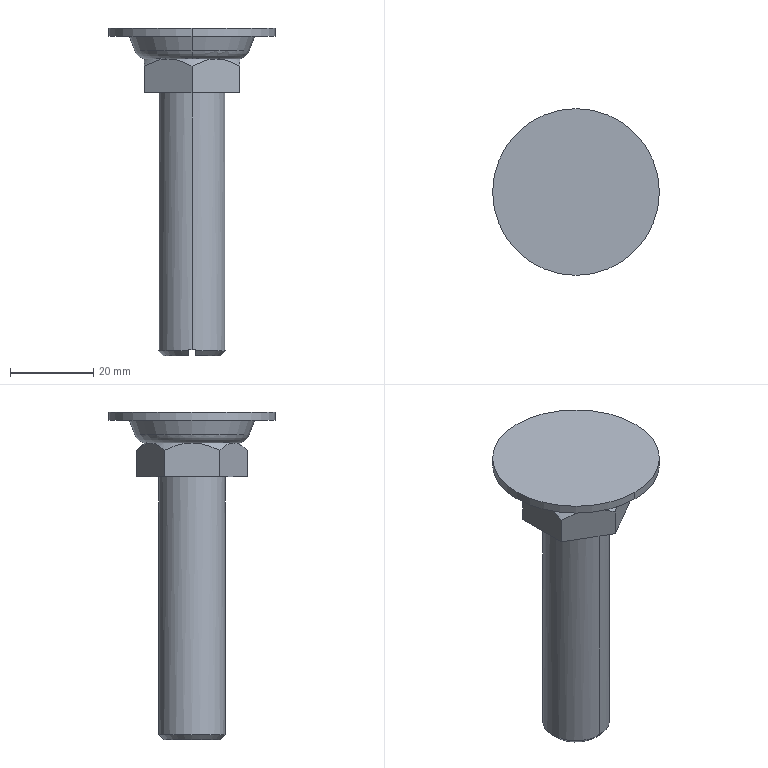Component | SolidWorks | CMAS50_F-2_CMAS50_Fadjuster-1 | 1 solid | 32 faces | box 40 x 40 x 78.6 mm | volume 22096 mm3 | plane 15 | cone 11 | cylinder 4 | torus 2 | commonest cylinder face diameters 16 x2 40 x2 | material 45
build123d program:
from build123d import *

# Parameters (mm, degrees)
SKETCH2_R           = 20
EXTRUDE1_DEPTH      = 11.47
EXTRUDE2_DEPTH      = 8
EXTRUDE2_DEPTH_BACK = 8
SKETCH3_W           = 1.5
SKETCH3_H           = 1.5


with BuildPart() as part:
    # Sketch1 → Revolve1 (revolve)
    with BuildSketch(Plane.XY, mode=Mode.PRIVATE) as revolve1_sk:
        with BuildLine():
            Line((0, 19.6), (6.773, 19.6))
            Line((6.773, 19.6), (8, 18.373))
            Line((8, 18.373), (8, -43.46))
            Line((8, -43.46), (15, -43.46))
            Line((15, -43.46), (15, -48.1))
            Line((15, -48.1), (11.5, -51.6))
            Line((11.5, -51.6), (10.912, -51.6))
            ThreePointArc((10.912, -51.6), (12.626, -52.138), (13.725, -53.558))
            Line((13.725, -53.558), (15, -57))
            Line((15, -57), (20, -57))
            Line((20, -57), (20, -59))
            Line((20, -59), (0, -59))
            Line((0, -59), (0, 19.6))
        make_face()
    revolve(revolve1_sk.sketch.rotate(Axis((0, -59, 0), (0, 1, 0)), 270), axis=Axis((0, -59, 0), (0, 1, 0)))

    # Sketch2 → Extrude1 (cut)
    with BuildSketch(Plane(origin=(0, -51.6, 0), x_dir=(1, 0, 0), z_dir=(0, 1, 0))):
        with Locations(Location((0, 0, 0), (0, 0, 270))):
            Circle(SKETCH2_R)
        Polygon((11.5, -6.64), (11.5, 6.64), (0, 13.279), (-11.5, 6.64), (-11.5, -6.64), (0, -13.279), align=None, mode=Mode.SUBTRACT)
    extrude(amount=EXTRUDE1_DEPTH, mode=Mode.SUBTRACT)

    # Sketch3 → Extrude2 (cut, two sides: drawn at the far end of the back side and taken through both)
    with BuildSketch(Plane.XY.offset(-EXTRUDE2_DEPTH_BACK)):
        with Locations((0, 18.85)):
            Rectangle(SKETCH3_W, SKETCH3_H)
    extrude(amount=EXTRUDE2_DEPTH + EXTRUDE2_DEPTH_BACK, mode=Mode.SUBTRACT)


solid = part.part

# Placed as in the assembly
solid = solid.moved(Location((264, 559, 620), (-90, 0, 0)))
STEP:
#1=COLOUR_RGB('',0.7922,0.8196,0.9333);
#2=FILL_AREA_STYLE_COLOUR('',#1);
#3=FILL_AREA_STYLE('',(#2));
#4=SURFACE_STYLE_FILL_AREA(#3);
#5=SURFACE_SIDE_STYLE('',(#4));
#6=SURFACE_STYLE_USAGE(.BOTH.,#5);
#7=PRESENTATION_STYLE_ASSIGNMENT((#6));
#8=CARTESIAN_POINT('',(10.394,22.323,26.12));
#9=VERTEX_POINT('',#8);
#10=CARTESIAN_POINT('',(10.394,21.693,26.12));
#11=VERTEX_POINT('',#10);
#12=CARTESIAN_POINT('',(10.394,22.008,26.12));
#13=DIRECTION('',(0.,0.,-1.));
#14=DIRECTION('',(0.,1.,0.));
#15=AXIS2_PLACEMENT_3D('',#12,#13,#14);
#16=CIRCLE('',#15,0.315);
#17=EDGE_CURVE('',#9,#11,#16,.T.);
#18=ORIENTED_EDGE('',*,*,#17,.T.);
#19=CARTESIAN_POINT('',(10.394,21.693,23.697));
#20=VERTEX_POINT('',#19);
#21=CARTESIAN_POINT('',(10.394,21.693,26.732));
#22=DIRECTION('',(0.,0.,-1.));
#23=VECTOR('',#22,39.37);
#24=LINE('',#21,#23);
#25=EDGE_CURVE('',#11,#20,#24,.T.);
#26=ORIENTED_EDGE('',*,*,#25,.T.);
#27=CARTESIAN_POINT('',(10.423,21.694,23.697));
#28=VERTEX_POINT('',#27);
#29=CARTESIAN_POINT('',(10.394,22.008,23.697));
#30=DIRECTION('',(0.,0.,1.));
#31=DIRECTION('',(0.,-1.,0.));
#32=AXIS2_PLACEMENT_3D('',#29,#30,#31);
#33=CIRCLE('',#32,0.315);
#34=EDGE_CURVE('',#20,#28,#33,.T.);
#35=ORIENTED_EDGE('',*,*,#34,.T.);
#36=CARTESIAN_POINT('',(10.423,21.694,23.686));
#37=VERTEX_POINT('',#36);
#38=CARTESIAN_POINT('',(10.423,21.694,26.732));
#39=DIRECTION('',(0.,0.,-1.));
#40=VECTOR('',#39,39.37);
#41=LINE('',#38,#40);
#42=EDGE_CURVE('',#28,#37,#41,.T.);
#43=ORIENTED_EDGE('',*,*,#42,.T.);
#44=CARTESIAN_POINT('',(10.423,22.321,23.686));
#45=VERTEX_POINT('',#44);
#46=CARTESIAN_POINT('',(10.394,22.008,23.686));
#47=DIRECTION('',(0.,0.,-1.));
#48=DIRECTION('',(0.,1.,0.));
#49=AXIS2_PLACEMENT_3D('',#46,#47,#48);
#50=CIRCLE('',#49,0.315);
#51=EDGE_CURVE('',#45,#37,#50,.T.);
#52=ORIENTED_EDGE('',*,*,#51,.F.);
#53=CARTESIAN_POINT('',(10.423,22.321,23.697));
#54=VERTEX_POINT('',#53);
#55=CARTESIAN_POINT('',(10.423,22.321,26.732));
#56=DIRECTION('',(0.,0.,1.));
#57=VECTOR('',#56,39.37);
#58=LINE('',#55,#57);
#59=EDGE_CURVE('',#45,#54,#58,.T.);
#60=ORIENTED_EDGE('',*,*,#59,.T.);
#61=CARTESIAN_POINT('',(10.394,22.323,23.697));
#62=VERTEX_POINT('',#61);
#63=CARTESIAN_POINT('',(10.394,22.008,23.697));
#64=DIRECTION('',(0.,0.,1.));
#65=DIRECTION('',(0.,-1.,0.));
#66=AXIS2_PLACEMENT_3D('',#63,#64,#65);
#67=CIRCLE('',#66,0.315);
#68=EDGE_CURVE('',#54,#62,#67,.T.);
#69=ORIENTED_EDGE('',*,*,#68,.T.);
#70=CARTESIAN_POINT('',(10.394,22.323,26.732));
#71=DIRECTION('',(0.,0.,-1.));
#72=VECTOR('',#71,39.37);
#73=LINE('',#70,#72);
#74=EDGE_CURVE('',#9,#62,#73,.T.);
#75=ORIENTED_EDGE('',*,*,#74,.F.);
#76=EDGE_LOOP('',(#18,#26,#35,#43,#52,#60,#69,#75));
#77=FACE_OUTER_BOUND('',#76,.T.);
#78=CARTESIAN_POINT('',(10.394,22.008,26.732));
#79=DIRECTION('',(0.,0.,-1.));
#80=DIRECTION('',(0.,1.,0.));
#81=AXIS2_PLACEMENT_3D('',#78,#79,#80);
#82=CYLINDRICAL_SURFACE('',#81,0.315);
#83=ADVANCED_FACE('',(#77),#82,.T.);
#84=CARTESIAN_POINT('',(10.394,22.795,26.732));
#85=VERTEX_POINT('',#84);
#86=CARTESIAN_POINT('',(10.394,21.22,26.732));
#87=VERTEX_POINT('',#86);
#88=CARTESIAN_POINT('',(10.394,22.008,26.732));
#89=DIRECTION('',(0.,0.,-1.));
#90=DIRECTION('',(0.,1.,0.));
#91=AXIS2_PLACEMENT_3D('',#88,#89,#90);
#92=CIRCLE('',#91,0.7874);
#93=EDGE_CURVE('',#85,#87,#92,.T.);
#94=ORIENTED_EDGE('',*,*,#93,.T.);
#95=CARTESIAN_POINT('',(10.394,21.22,26.654));
#96=VERTEX_POINT('',#95);
#97=CARTESIAN_POINT('',(10.394,21.22,26.732));
#98=DIRECTION('',(0.,0.,-1.));
#99=VECTOR('',#98,39.37);
#100=LINE('',#97,#99);
#101=EDGE_CURVE('',#87,#96,#100,.T.);
#102=ORIENTED_EDGE('',*,*,#101,.T.);
#103=CARTESIAN_POINT('',(10.394,22.795,26.654));
#104=VERTEX_POINT('',#103);
#105=CARTESIAN_POINT('',(10.394,22.008,26.654));
#106=DIRECTION('',(0.,0.,-1.));
#107=DIRECTION('',(0.,1.,0.));
#108=AXIS2_PLACEMENT_3D('',#105,#106,#107);
#109=CIRCLE('',#108,0.7874);
#110=EDGE_CURVE('',#104,#96,#109,.T.);
#111=ORIENTED_EDGE('',*,*,#110,.F.);
#112=CARTESIAN_POINT('',(10.394,22.795,26.732));
#113=DIRECTION('',(0.,0.,-1.));
#114=VECTOR('',#113,39.37);
#115=LINE('',#112,#114);
#116=EDGE_CURVE('',#85,#104,#115,.T.);
#117=ORIENTED_EDGE('',*,*,#116,.F.);
#118=EDGE_LOOP('',(#94,#102,#111,#117));
#119=FACE_OUTER_BOUND('',#118,.T.);
#120=CARTESIAN_POINT('',(10.394,22.008,26.732));
#121=DIRECTION('',(0.,0.,-1.));
#122=DIRECTION('',(0.,1.,0.));
#123=AXIS2_PLACEMENT_3D('',#120,#121,#122);
#124=CYLINDRICAL_SURFACE('',#123,0.7874);
#125=ADVANCED_FACE('',(#119),#124,.T.);
#126=CARTESIAN_POINT('',(10.394,22.548,26.518));
#127=VERTEX_POINT('',#126);
#128=CARTESIAN_POINT('',(10.394,21.468,26.518));
#129=VERTEX_POINT('',#128);
#130=CARTESIAN_POINT('',(10.394,22.008,26.518));
#131=DIRECTION('',(0.,0.,-1.));
#132=DIRECTION('',(0.,1.,0.));
#133=AXIS2_PLACEMENT_3D('',#130,#131,#132);
#134=CIRCLE('',#133,0.5404);
#135=EDGE_CURVE('',#127,#129,#134,.T.);
#136=ORIENTED_EDGE('',*,*,#135,.F.);
#137=CARTESIAN_POINT('',(10.394,22.598,26.654));
#138=VERTEX_POINT('',#137);
#139=CARTESIAN_POINT('',(10.394,22.598,26.654));
#140=DIRECTION('',(0.,0.3473,0.9377));
#141=VECTOR('',#140,39.37);
#142=LINE('',#139,#141);
#143=EDGE_CURVE('',#127,#138,#142,.T.);
#144=ORIENTED_EDGE('',*,*,#143,.T.);
#145=CARTESIAN_POINT('',(10.394,21.417,26.654));
#146=VERTEX_POINT('',#145);
#147=CARTESIAN_POINT('',(10.394,22.008,26.654));
#148=DIRECTION('',(0.,0.,-1.));
#149=DIRECTION('',(0.,1.,0.));
#150=AXIS2_PLACEMENT_3D('',#147,#148,#149);
#151=CIRCLE('',#150,0.5906);
#152=EDGE_CURVE('',#138,#146,#151,.T.);
#153=ORIENTED_EDGE('',*,*,#152,.T.);
#154=CARTESIAN_POINT('',(10.394,21.417,26.654));
#155=DIRECTION('',(0.,-0.3473,0.9377));
#156=VECTOR('',#155,39.37);
#157=LINE('',#154,#156);
#158=EDGE_CURVE('',#129,#146,#157,.T.);
#159=ORIENTED_EDGE('',*,*,#158,.F.);
#160=EDGE_LOOP('',(#136,#144,#153,#159));
#161=FACE_OUTER_BOUND('',#160,.T.);
#162=CARTESIAN_POINT('',(10.394,22.008,26.654));
#163=DIRECTION('',(0.,0.,1.));
#164=DIRECTION('',(0.,-1.,0.));
#165=AXIS2_PLACEMENT_3D('',#162,#163,#164);
#166=CONICAL_SURFACE('',#165,0.5906,0.3547);
#167=ADVANCED_FACE('',(#161),#166,.T.);
#168=ORIENTED_EDGE('',*,*,#135,.T.);
#169=CARTESIAN_POINT('',(10.394,21.578,26.441));
#170=VERTEX_POINT('',#169);
#171=CARTESIAN_POINT('',(10.394,21.578,26.559));
#172=DIRECTION('',(1.,0.,0.));
#173=DIRECTION('',(0.,1.,0.));
#174=AXIS2_PLACEMENT_3D('',#171,#172,#173);
#175=CIRCLE('',#174,0.1181);
#176=EDGE_CURVE('',#129,#170,#175,.T.);
#177=ORIENTED_EDGE('',*,*,#176,.T.);
#178=CARTESIAN_POINT('',(10.394,22.437,26.441));
#179=VERTEX_POINT('',#178);
#180=CARTESIAN_POINT('',(10.394,22.008,26.441));
#181=DIRECTION('',(0.,0.,-1.));
#182=DIRECTION('',(0.,1.,0.));
#183=AXIS2_PLACEMENT_3D('',#180,#181,#182);
#184=CIRCLE('',#183,0.4296);
#185=EDGE_CURVE('',#179,#170,#184,.T.);
#186=ORIENTED_EDGE('',*,*,#185,.F.);
#187=CARTESIAN_POINT('',(10.394,22.437,26.559));
#188=DIRECTION('',(-1.,0.,0.));
#189=DIRECTION('',(0.,0.,1.));
#190=AXIS2_PLACEMENT_3D('',#187,#188,#189);
#191=CIRCLE('',#190,0.1181);
#192=EDGE_CURVE('',#127,#179,#191,.T.);
#193=ORIENTED_EDGE('',*,*,#192,.F.);
#194=EDGE_LOOP('',(#168,#177,#186,#193));
#195=FACE_OUTER_BOUND('',#194,.T.);
#196=CARTESIAN_POINT('',(10.394,22.008,26.559));
#197=DIRECTION('',(0.,0.,-1.));
#198=DIRECTION('',(0.,1.,0.));
#199=AXIS2_PLACEMENT_3D('',#196,#197,#198);
#200=TOROIDAL_SURFACE('',#199,0.4296,0.1181);
#201=ADVANCED_FACE('',(#195),#200,.T.);
#202=CARTESIAN_POINT('',(10.167,22.4,26.441));
#203=VERTEX_POINT('',#202);
#204=CARTESIAN_POINT('',(10.394,22.461,26.441));
#205=VERTEX_POINT('',#204);
#206=CARTESIAN_POINT('',(10.394,22.008,26.441));
#207=DIRECTION('',(0.,0.,-1.));
#208=DIRECTION('',(0.,1.,0.));
#209=AXIS2_PLACEMENT_3D('',#206,#207,#208);
#210=CIRCLE('',#209,0.4528);
#211=EDGE_CURVE('',#203,#205,#210,.T.);
#212=ORIENTED_EDGE('',*,*,#211,.T.);
#213=CARTESIAN_POINT('',(10.394,22.531,26.371));
#214=VERTEX_POINT('',#213);
#215=CARTESIAN_POINT('',(10.394,22.461,26.441));
#216=DIRECTION('',(0.,0.7071,-0.7071));
#217=VECTOR('',#216,39.37);
#218=LINE('',#215,#217);
#219=EDGE_CURVE('',#205,#214,#218,.T.);
#220=ORIENTED_EDGE('',*,*,#219,.T.);
#221=CARTESIAN_POINT('',(10.394,22.531,26.371));
#222=CARTESIAN_POINT('',(10.358,22.51,26.391));
#223=CARTESIAN_POINT('',(10.322,22.489,26.409));
#224=CARTESIAN_POINT('',(10.265,22.457,26.427));
#225=CARTESIAN_POINT('',(10.246,22.446,26.432));
#226=CARTESIAN_POINT('',(10.207,22.423,26.439));
#227=CARTESIAN_POINT('',(10.187,22.411,26.441));
#228=CARTESIAN_POINT('',(10.167,22.4,26.441));
#229=B_SPLINE_CURVE_WITH_KNOTS('',3,(#221,#222,#223,#224,#225,#226,#227,#228),.UNSPECIFIED.,.F.,.F.,(4,2,2,4),(0.00000025,0.003441,0.005162,0.006883),.UNSPECIFIED.);
#230=EDGE_CURVE('',#214,#203,#229,.T.);
#231=ORIENTED_EDGE('',*,*,#230,.T.);
#232=EDGE_LOOP('',(#212,#220,#231));
#233=FACE_OUTER_BOUND('',#232,.T.);
#234=CARTESIAN_POINT('',(10.394,22.008,26.441));
#235=DIRECTION('',(0.,0.,-1.));
#236=DIRECTION('',(0.,1.,0.));
#237=AXIS2_PLACEMENT_3D('',#234,#235,#236);
#238=CONICAL_SURFACE('',#237,0.4528,0.7854);
#239=ADVANCED_FACE('',(#233),#238,.T.);
#240=CARTESIAN_POINT('',(10.364,21.743,23.638));
#241=VERTEX_POINT('',#240);
#242=CARTESIAN_POINT('',(10.364,22.273,23.638));
#243=VERTEX_POINT('',#242);
#244=CARTESIAN_POINT('',(10.394,22.008,23.638));
#245=DIRECTION('',(0.,0.,-1.));
#246=DIRECTION('',(0.,1.,0.));
#247=AXIS2_PLACEMENT_3D('',#244,#245,#246);
#248=CIRCLE('',#247,0.2667);
#249=EDGE_CURVE('',#241,#243,#248,.T.);
#250=ORIENTED_EDGE('',*,*,#249,.T.);
#251=CARTESIAN_POINT('',(10.364,21.693,23.638));
#252=DIRECTION('',(0.,1.,0.));
#253=VECTOR('',#252,39.37);
#254=LINE('',#251,#253);
#255=EDGE_CURVE('',#241,#243,#254,.T.);
#256=ORIENTED_EDGE('',*,*,#255,.F.);
#257=EDGE_LOOP('',(#250,#256));
#258=FACE_OUTER_BOUND('',#257,.T.);
#259=CARTESIAN_POINT('',(10.394,22.008,23.638));
#260=DIRECTION('',(0.,0.,1.));
#261=DIRECTION('',(0.,-1.,0.));
#262=AXIS2_PLACEMENT_3D('',#259,#260,#261);
#263=PLANE('',#262);
#264=ADVANCED_FACE('',(#258),#263,.F.);
#265=CARTESIAN_POINT('',(10.364,21.694,23.686));
#266=VERTEX_POINT('',#265);
#267=CARTESIAN_POINT('',(10.364,22.321,23.686));
#268=VERTEX_POINT('',#267);
#269=CARTESIAN_POINT('',(10.394,22.008,23.686));
#270=DIRECTION('',(0.,0.,-1.));
#271=DIRECTION('',(0.,1.,0.));
#272=AXIS2_PLACEMENT_3D('',#269,#270,#271);
#273=CIRCLE('',#272,0.315);
#274=EDGE_CURVE('',#266,#268,#273,.T.);
#275=ORIENTED_EDGE('',*,*,#274,.T.);
#276=CARTESIAN_POINT('',(10.364,22.321,23.686));
#277=CARTESIAN_POINT('',(10.364,22.305,23.67));
#278=CARTESIAN_POINT('',(10.364,22.289,23.654));
#279=CARTESIAN_POINT('',(10.364,22.273,23.638));
#280=B_SPLINE_CURVE_WITH_KNOTS('',3,(#276,#277,#278,#279),.UNSPECIFIED.,.F.,.F.,(4,4),(0.01363,0.01537),.UNSPECIFIED.);
#281=EDGE_CURVE('',#268,#243,#280,.T.);
#282=ORIENTED_EDGE('',*,*,#281,.T.);
#283=ORIENTED_EDGE('',*,*,#249,.F.);
#284=CARTESIAN_POINT('',(10.364,21.743,23.638));
#285=CARTESIAN_POINT('',(10.364,21.727,23.654));
#286=CARTESIAN_POINT('',(10.364,21.71,23.67));
#287=CARTESIAN_POINT('',(10.364,21.694,23.686));
#288=B_SPLINE_CURVE_WITH_KNOTS('',3,(#284,#285,#286,#287),.UNSPECIFIED.,.F.,.F.,(4,4),(0.03362,0.03537),.UNSPECIFIED.);
#289=EDGE_CURVE('',#241,#266,#288,.T.);
#290=ORIENTED_EDGE('',*,*,#289,.T.);
#291=EDGE_LOOP('',(#275,#282,#283,#290));
#292=FACE_OUTER_BOUND('',#291,.T.);
#293=CARTESIAN_POINT('',(10.394,22.008,23.686));
#294=DIRECTION('',(0.,0.,1.));
#295=DIRECTION('',(0.,-1.,0.));
#296=AXIS2_PLACEMENT_3D('',#293,#294,#295);
#297=CONICAL_SURFACE('',#296,0.315,0.7854);
#298=ADVANCED_FACE('',(#292),#297,.T.);
#299=CARTESIAN_POINT('',(10.167,21.616,26.441));
#300=VERTEX_POINT('',#299);
#301=CARTESIAN_POINT('',(10.394,21.485,26.371));
#302=VERTEX_POINT('',#301);
#303=CARTESIAN_POINT('',(10.167,21.616,26.441));
#304=CARTESIAN_POINT('',(10.207,21.593,26.441));
#305=CARTESIAN_POINT('',(10.245,21.571,26.434));
#306=CARTESIAN_POINT('',(10.322,21.527,26.409));
#307=CARTESIAN_POINT('',(10.358,21.506,26.391));
#308=CARTESIAN_POINT('',(10.394,21.485,26.371));
#309=B_SPLINE_CURVE_WITH_KNOTS('',3,(#303,#304,#305,#306,#307,#308),.UNSPECIFIED.,.F.,.F.,(4,2,4),(0.006883,0.0103,0.01372),.UNSPECIFIED.);
#310=EDGE_CURVE('',#300,#302,#309,.T.);
#311=ORIENTED_EDGE('',*,*,#310,.T.);
#312=CARTESIAN_POINT('',(10.62,21.616,26.441));
#313=VERTEX_POINT('',#312);
#314=CARTESIAN_POINT('',(10.394,21.485,26.371));
#315=CARTESIAN_POINT('',(10.429,21.506,26.391));
#316=CARTESIAN_POINT('',(10.466,21.527,26.409));
#317=CARTESIAN_POINT('',(10.522,21.559,26.427));
#318=CARTESIAN_POINT('',(10.541,21.57,26.432));
#319=CARTESIAN_POINT('',(10.58,21.593,26.439));
#320=CARTESIAN_POINT('',(10.6,21.604,26.441));
#321=CARTESIAN_POINT('',(10.62,21.616,26.441));
#322=B_SPLINE_CURVE_WITH_KNOTS('',3,(#314,#315,#316,#317,#318,#319,#320,#321),.UNSPECIFIED.,.F.,.F.,(4,2,2,4),(0.00000025,0.003441,0.005162,0.006883),.UNSPECIFIED.);
#323=EDGE_CURVE('',#302,#313,#322,.T.);
#324=ORIENTED_EDGE('',*,*,#323,.T.);
#325=CARTESIAN_POINT('',(10.394,22.008,26.441));
#326=DIRECTION('',(0.,0.,-1.));
#327=DIRECTION('',(0.,1.,0.));
#328=AXIS2_PLACEMENT_3D('',#325,#326,#327);
#329=CIRCLE('',#328,0.4528);
#330=EDGE_CURVE('',#313,#300,#329,.T.);
#331=ORIENTED_EDGE('',*,*,#330,.T.);
#332=EDGE_LOOP('',(#311,#324,#331));
#333=FACE_OUTER_BOUND('',#332,.T.);
#334=CARTESIAN_POINT('',(10.394,22.008,26.441));
#335=DIRECTION('',(0.,0.,-1.));
#336=DIRECTION('',(0.,1.,0.));
#337=AXIS2_PLACEMENT_3D('',#334,#335,#336);
#338=CONICAL_SURFACE('',#337,0.4528,0.7854);
#339=ADVANCED_FACE('',(#333),#338,.T.);
#340=CARTESIAN_POINT('',(10.846,22.008,26.441));
#341=VERTEX_POINT('',#340);
#342=CARTESIAN_POINT('',(10.394,22.008,26.441));
#343=DIRECTION('',(0.,0.,-1.));
#344=DIRECTION('',(0.,1.,0.));
#345=AXIS2_PLACEMENT_3D('',#342,#343,#344);
#346=CIRCLE('',#345,0.4528);
#347=EDGE_CURVE('',#341,#313,#346,.T.);
#348=ORIENTED_EDGE('',*,*,#347,.T.);
#349=CARTESIAN_POINT('',(10.846,21.746,26.371));
#350=VERTEX_POINT('',#349);
#351=CARTESIAN_POINT('',(10.62,21.616,26.441));
#352=CARTESIAN_POINT('',(10.659,21.639,26.441));
#353=CARTESIAN_POINT('',(10.698,21.661,26.434));
#354=CARTESIAN_POINT('',(10.775,21.705,26.409));
#355=CARTESIAN_POINT('',(10.811,21.726,26.391));
#356=CARTESIAN_POINT('',(10.846,21.746,26.371));
#357=B_SPLINE_CURVE_WITH_KNOTS('',3,(#351,#352,#353,#354,#355,#356),.UNSPECIFIED.,.F.,.F.,(4,2,4),(0.006883,0.0103,0.01372),.UNSPECIFIED.);
#358=EDGE_CURVE('',#313,#350,#357,.T.);
#359=ORIENTED_EDGE('',*,*,#358,.T.);
#360=CARTESIAN_POINT('',(10.846,21.746,26.371));
#361=CARTESIAN_POINT('',(10.846,21.767,26.381));
#362=CARTESIAN_POINT('',(10.846,21.788,26.391));
#363=CARTESIAN_POINT('',(10.846,21.83,26.408));
#364=CARTESIAN_POINT('',(10.846,21.851,26.415));
#365=CARTESIAN_POINT('',(10.846,21.895,26.428));
#366=CARTESIAN_POINT('',(10.846,21.917,26.432));
#367=CARTESIAN_POINT('',(10.846,21.951,26.437));
#368=CARTESIAN_POINT('',(10.846,21.962,26.439));
#369=CARTESIAN_POINT('',(10.846,21.985,26.441));
#370=CARTESIAN_POINT('',(10.846,21.996,26.441));
#371=CARTESIAN_POINT('',(10.846,22.008,26.441));
#372=B_SPLINE_CURVE_WITH_KNOTS('',3,(#360,#361,#362,#363,#364,#365,#366,#367,#368,#369,#370,#371),.UNSPECIFIED.,.F.,.F.,(4,2,2,2,2,4),(0.01208,0.0138,0.01551,0.01723,0.01808,0.01894),.UNSPECIFIED.);
#373=EDGE_CURVE('',#350,#341,#372,.T.);
#374=ORIENTED_EDGE('',*,*,#373,.T.);
#375=EDGE_LOOP('',(#348,#359,#374));
#376=FACE_OUTER_BOUND('',#375,.T.);
#377=CARTESIAN_POINT('',(10.394,22.008,26.441));
#378=DIRECTION('',(0.,0.,-1.));
#379=DIRECTION('',(0.,1.,0.));
#380=AXIS2_PLACEMENT_3D('',#377,#378,#379);
#381=CONICAL_SURFACE('',#380,0.4528,0.7854);
#382=ADVANCED_FACE('',(#376),#381,.T.);
#383=CARTESIAN_POINT('',(10.62,22.4,26.441));
#384=VERTEX_POINT('',#383);
#385=CARTESIAN_POINT('',(10.394,22.008,26.441));
#386=DIRECTION('',(0.,0.,-1.));
#387=DIRECTION('',(0.,1.,0.));
#388=AXIS2_PLACEMENT_3D('',#385,#386,#387);
#389=CIRCLE('',#388,0.4528);
#390=EDGE_CURVE('',#384,#341,#389,.T.);
#391=ORIENTED_EDGE('',*,*,#390,.T.);
#392=CARTESIAN_POINT('',(10.846,22.269,26.371));
#393=VERTEX_POINT('',#392);
#394=CARTESIAN_POINT('',(10.846,22.008,26.441));
#395=CARTESIAN_POINT('',(10.846,22.054,26.441));
#396=CARTESIAN_POINT('',(10.846,22.099,26.434));
#397=CARTESIAN_POINT('',(10.846,22.164,26.415));
#398=CARTESIAN_POINT('',(10.846,22.186,26.408));
#399=CARTESIAN_POINT('',(10.846,22.228,26.39));
#400=CARTESIAN_POINT('',(10.846,22.249,26.381));
#401=CARTESIAN_POINT('',(10.846,22.269,26.371));
#402=B_SPLINE_CURVE_WITH_KNOTS('',3,(#394,#395,#396,#397,#398,#399,#400,#401),.UNSPECIFIED.,.F.,.F.,(4,2,2,4),(0.01894,0.02237,0.02409,0.0258),.UNSPECIFIED.);
#403=EDGE_CURVE('',#341,#393,#402,.T.);
#404=ORIENTED_EDGE('',*,*,#403,.T.);
#405=CARTESIAN_POINT('',(10.846,22.269,26.371));
#406=CARTESIAN_POINT('',(10.811,22.29,26.391));
#407=CARTESIAN_POINT('',(10.775,22.311,26.409));
#408=CARTESIAN_POINT('',(10.718,22.343,26.427));
#409=CARTESIAN_POINT('',(10.699,22.354,26.432));
#410=CARTESIAN_POINT('',(10.66,22.377,26.439));
#411=CARTESIAN_POINT('',(10.64,22.389,26.441));
#412=CARTESIAN_POINT('',(10.62,22.4,26.441));
#413=B_SPLINE_CURVE_WITH_KNOTS('',3,(#405,#406,#407,#408,#409,#410,#411,#412),.UNSPECIFIED.,.F.,.F.,(4,2,2,4),(0.00000025,0.003441,0.005162,0.006883),.UNSPECIFIED.);
#414=EDGE_CURVE('',#393,#384,#413,.T.);
#415=ORIENTED_EDGE('',*,*,#414,.T.);
#416=EDGE_LOOP('',(#391,#404,#415));
#417=FACE_OUTER_BOUND('',#416,.T.);
#418=CARTESIAN_POINT('',(10.394,22.008,26.441));
#419=DIRECTION('',(0.,0.,-1.));
#420=DIRECTION('',(0.,1.,0.));
#421=AXIS2_PLACEMENT_3D('',#418,#419,#420);
#422=CONICAL_SURFACE('',#421,0.4528,0.7854);
#423=ADVANCED_FACE('',(#417),#422,.T.);
#424=CARTESIAN_POINT('',(9.941,22.008,26.441));
#425=VERTEX_POINT('',#424);
#426=CARTESIAN_POINT('',(9.941,21.746,26.371));
#427=VERTEX_POINT('',#426);
#428=CARTESIAN_POINT('',(9.941,22.008,26.441));
#429=CARTESIAN_POINT('',(9.941,21.996,26.441));
#430=CARTESIAN_POINT('',(9.941,21.985,26.441));
#431=CARTESIAN_POINT('',(9.941,21.962,26.439));
#432=CARTESIAN_POINT('',(9.941,21.928,26.435));
#433=CARTESIAN_POINT('',(9.941,21.895,26.428));
#434=CARTESIAN_POINT('',(9.941,21.851,26.415));
#435=CARTESIAN_POINT('',(9.941,21.83,26.408));
#436=CARTESIAN_POINT('',(9.941,21.788,26.391));
#437=CARTESIAN_POINT('',(9.941,21.767,26.381));
#438=CARTESIAN_POINT('',(9.941,21.746,26.371));
#439=B_SPLINE_CURVE_WITH_KNOTS('',3,(#428,#429,#430,#431,#432,#433,#434,#435,#436,#437,#438),.UNSPECIFIED.,.F.,.F.,(4,2,1,2,2,4),(0.01385,0.01471,0.01557,0.01729,0.01901,0.02073),.UNSPECIFIED.);
#440=EDGE_CURVE('',#425,#427,#439,.T.);
#441=ORIENTED_EDGE('',*,*,#440,.T.);
#442=CARTESIAN_POINT('',(9.941,21.746,26.371));
#443=CARTESIAN_POINT('',(9.976,21.726,26.391));
#444=CARTESIAN_POINT('',(10.013,21.705,26.409));
#445=CARTESIAN_POINT('',(10.069,21.672,26.427));
#446=CARTESIAN_POINT('',(10.088,21.661,26.432));
#447=CARTESIAN_POINT('',(10.127,21.639,26.439));
#448=CARTESIAN_POINT('',(10.147,21.627,26.441));
#449=CARTESIAN_POINT('',(10.167,21.616,26.441));
#450=B_SPLINE_CURVE_WITH_KNOTS('',3,(#442,#443,#444,#445,#446,#447,#448,#449),.UNSPECIFIED.,.F.,.F.,(4,2,2,4),(0.00000025,0.003441,0.005162,0.006883),.UNSPECIFIED.);
#451=EDGE_CURVE('',#427,#300,#450,.T.);
#452=ORIENTED_EDGE('',*,*,#451,.T.);
#453=CARTESIAN_POINT('',(10.394,22.008,26.441));
#454=DIRECTION('',(0.,0.,-1.));
#455=DIRECTION('',(0.,1.,0.));
#456=AXIS2_PLACEMENT_3D('',#453,#454,#455);
#457=CIRCLE('',#456,0.4528);
#458=EDGE_CURVE('',#300,#425,#457,.T.);
#459=ORIENTED_EDGE('',*,*,#458,.T.);
#460=EDGE_LOOP('',(#441,#452,#459));
#461=FACE_OUTER_BOUND('',#460,.T.);
#462=CARTESIAN_POINT('',(10.394,22.008,26.441));
#463=DIRECTION('',(0.,0.,-1.));
#464=DIRECTION('',(0.,1.,0.));
#465=AXIS2_PLACEMENT_3D('',#462,#463,#464);
#466=CONICAL_SURFACE('',#465,0.4528,0.7854);
#467=ADVANCED_FACE('',(#461),#466,.T.);
#468=ORIENTED_EDGE('',*,*,#219,.F.);
#469=CARTESIAN_POINT('',(10.394,22.008,26.441));
#470=DIRECTION('',(0.,0.,-1.));
#471=DIRECTION('',(0.,1.,0.));
#472=AXIS2_PLACEMENT_3D('',#469,#470,#471);
#473=CIRCLE('',#472,0.4528);
#474=EDGE_CURVE('',#205,#384,#473,.T.);
#475=ORIENTED_EDGE('',*,*,#474,.T.);
#476=CARTESIAN_POINT('',(10.62,22.4,26.441));
#477=CARTESIAN_POINT('',(10.581,22.423,26.441));
#478=CARTESIAN_POINT('',(10.542,22.445,26.434));
#479=CARTESIAN_POINT('',(10.466,22.489,26.409));
#480=CARTESIAN_POINT('',(10.429,22.51,26.391));
#481=CARTESIAN_POINT('',(10.394,22.531,26.371));
#482=B_SPLINE_CURVE_WITH_KNOTS('',3,(#476,#477,#478,#479,#480,#481),.UNSPECIFIED.,.F.,.F.,(4,2,4),(0.006883,0.0103,0.01372),.UNSPECIFIED.);
#483=EDGE_CURVE('',#384,#214,#482,.T.);
#484=ORIENTED_EDGE('',*,*,#483,.T.);
#485=EDGE_LOOP('',(#468,#475,#484));
#486=FACE_OUTER_BOUND('',#485,.T.);
#487=CARTESIAN_POINT('',(10.394,22.008,26.441));
#488=DIRECTION('',(0.,0.,-1.));
#489=DIRECTION('',(0.,1.,0.));
#490=AXIS2_PLACEMENT_3D('',#487,#488,#489);
#491=CONICAL_SURFACE('',#490,0.4528,0.7854);
#492=ADVANCED_FACE('',(#486),#491,.T.);
#493=CARTESIAN_POINT('',(9.941,22.269,26.371));
#494=VERTEX_POINT('',#493);
#495=CARTESIAN_POINT('',(10.167,22.4,26.441));
#496=CARTESIAN_POINT('',(10.128,22.377,26.441));
#497=CARTESIAN_POINT('',(10.089,22.355,26.434));
#498=CARTESIAN_POINT('',(10.013,22.311,26.409));
#499=CARTESIAN_POINT('',(9.976,22.29,26.391));
#500=CARTESIAN_POINT('',(9.941,22.269,26.371));
#501=B_SPLINE_CURVE_WITH_KNOTS('',3,(#495,#496,#497,#498,#499,#500),.UNSPECIFIED.,.F.,.F.,(4,2,4),(0.006883,0.0103,0.01372),.UNSPECIFIED.);
#502=EDGE_CURVE('',#203,#494,#501,.T.);
#503=ORIENTED_EDGE('',*,*,#502,.T.);
#504=CARTESIAN_POINT('',(9.941,22.269,26.371));
#505=CARTESIAN_POINT('',(9.941,22.249,26.381));
#506=CARTESIAN_POINT('',(9.941,22.228,26.39));
#507=CARTESIAN_POINT('',(9.941,22.186,26.408));
#508=CARTESIAN_POINT('',(9.941,22.164,26.415));
#509=CARTESIAN_POINT('',(9.941,22.099,26.434));
#510=CARTESIAN_POINT('',(9.941,22.054,26.441));
#511=CARTESIAN_POINT('',(9.941,22.008,26.441));
#512=B_SPLINE_CURVE_WITH_KNOTS('',3,(#504,#505,#506,#507,#508,#509,#510,#511),.UNSPECIFIED.,.F.,.F.,(4,2,2,4),(0.006963,0.008685,0.01041,0.01385),.UNSPECIFIED.);
#513=EDGE_CURVE('',#494,#425,#512,.T.);
#514=ORIENTED_EDGE('',*,*,#513,.T.);
#515=CARTESIAN_POINT('',(10.394,22.008,26.441));
#516=DIRECTION('',(0.,0.,-1.));
#517=DIRECTION('',(0.,1.,0.));
#518=AXIS2_PLACEMENT_3D('',#515,#516,#517);
#519=CIRCLE('',#518,0.4528);
#520=EDGE_CURVE('',#425,#203,#519,.T.);
#521=ORIENTED_EDGE('',*,*,#520,.T.);
#522=EDGE_LOOP('',(#503,#514,#521));
#523=FACE_OUTER_BOUND('',#522,.T.);
#524=CARTESIAN_POINT('',(10.394,22.008,26.441));
#525=DIRECTION('',(0.,0.,-1.));
#526=DIRECTION('',(0.,1.,0.));
#527=AXIS2_PLACEMENT_3D('',#524,#525,#526);
#528=CONICAL_SURFACE('',#527,0.4528,0.7854);
#529=ADVANCED_FACE('',(#523),#528,.T.);
#530=ORIENTED_EDGE('',*,*,#390,.F.);
#531=ORIENTED_EDGE('',*,*,#474,.F.);
#532=ORIENTED_EDGE('',*,*,#211,.F.);
#533=ORIENTED_EDGE('',*,*,#520,.F.);
#534=ORIENTED_EDGE('',*,*,#458,.F.);
#535=ORIENTED_EDGE('',*,*,#330,.F.);
#536=ORIENTED_EDGE('',*,*,#347,.F.);
#537=EDGE_LOOP('',(#530,#531,#532,#533,#534,#535,#536));
#538=FACE_OUTER_BOUND('',#537,.T.);
#539=ORIENTED_EDGE('',*,*,#185,.T.);
#540=CARTESIAN_POINT('',(10.394,22.008,26.441));
#541=DIRECTION('',(0.,0.,-1.));
#542=DIRECTION('',(0.,1.,0.));
#543=AXIS2_PLACEMENT_3D('',#540,#541,#542);
#544=CIRCLE('',#543,0.4296);
#545=EDGE_CURVE('',#170,#179,#544,.T.);
#546=ORIENTED_EDGE('',*,*,#545,.T.);
#547=EDGE_LOOP('',(#539,#546));
#548=FACE_BOUND('',#547,.T.);
#549=CARTESIAN_POINT('',(10.846,22.008,26.441));
#550=DIRECTION('',(0.,0.,-1.));
#551=DIRECTION('',(0.,1.,0.));
#552=AXIS2_PLACEMENT_3D('',#549,#550,#551);
#553=PLANE('',#552);
#554=ADVANCED_FACE('',(#538,#548),#553,.F.);
#555=ORIENTED_EDGE('',*,*,#176,.F.);
#556=CARTESIAN_POINT('',(10.394,22.008,26.518));
#557=DIRECTION('',(0.,0.,-1.));
#558=DIRECTION('',(0.,1.,0.));
#559=AXIS2_PLACEMENT_3D('',#556,#557,#558);
#560=CIRCLE('',#559,0.5404);
#561=EDGE_CURVE('',#129,#127,#560,.T.);
#562=ORIENTED_EDGE('',*,*,#561,.T.);
#563=ORIENTED_EDGE('',*,*,#192,.T.);
#564=ORIENTED_EDGE('',*,*,#545,.F.);
#565=EDGE_LOOP('',(#555,#562,#563,#564));
#566=FACE_OUTER_BOUND('',#565,.T.);
#567=CARTESIAN_POINT('',(10.394,22.008,26.559));
#568=DIRECTION('',(0.,0.,-1.));
#569=DIRECTION('',(0.,1.,0.));
#570=AXIS2_PLACEMENT_3D('',#567,#568,#569);
#571=TOROIDAL_SURFACE('',#570,0.4296,0.1181);
#572=ADVANCED_FACE('',(#566),#571,.T.);
#573=ORIENTED_EDGE('',*,*,#143,.F.);
#574=ORIENTED_EDGE('',*,*,#561,.F.);
#575=ORIENTED_EDGE('',*,*,#158,.T.);
#576=CARTESIAN_POINT('',(10.394,22.008,26.654));
#577=DIRECTION('',(0.,0.,-1.));
#578=DIRECTION('',(0.,1.,0.));
#579=AXIS2_PLACEMENT_3D('',#576,#577,#578);
#580=CIRCLE('',#579,0.5906);
#581=EDGE_CURVE('',#146,#138,#580,.T.);
#582=ORIENTED_EDGE('',*,*,#581,.T.);
#583=EDGE_LOOP('',(#573,#574,#575,#582));
#584=FACE_OUTER_BOUND('',#583,.T.);
#585=CARTESIAN_POINT('',(10.394,22.008,26.654));
#586=DIRECTION('',(0.,0.,1.));
#587=DIRECTION('',(0.,-1.,0.));
#588=AXIS2_PLACEMENT_3D('',#585,#586,#587);
#589=CONICAL_SURFACE('',#588,0.5906,0.3547);
#590=ADVANCED_FACE('',(#584),#589,.T.);
#591=ORIENTED_EDGE('',*,*,#581,.F.);
#592=ORIENTED_EDGE('',*,*,#152,.F.);
#593=EDGE_LOOP('',(#591,#592));
#594=FACE_BOUND('',#593,.T.);
#595=ORIENTED_EDGE('',*,*,#110,.T.);
#596=CARTESIAN_POINT('',(10.394,22.008,26.654));
#597=DIRECTION('',(0.,0.,-1.));
#598=DIRECTION('',(0.,1.,0.));
#599=AXIS2_PLACEMENT_3D('',#596,#597,#598);
#600=CIRCLE('',#599,0.7874);
#601=EDGE_CURVE('',#96,#104,#600,.T.);
#602=ORIENTED_EDGE('',*,*,#601,.T.);
#603=EDGE_LOOP('',(#595,#602));
#604=FACE_OUTER_BOUND('',#603,.T.);
#605=CARTESIAN_POINT('',(10.984,22.008,26.654));
#606=DIRECTION('',(0.,0.,1.));
#607=DIRECTION('',(0.,-1.,0.));
#608=AXIS2_PLACEMENT_3D('',#605,#606,#607);
#609=PLANE('',#608);
#610=ADVANCED_FACE('',(#594,#604),#609,.F.);
#611=ORIENTED_EDGE('',*,*,#101,.F.);
#612=CARTESIAN_POINT('',(10.394,22.008,26.732));
#613=DIRECTION('',(0.,0.,-1.));
#614=DIRECTION('',(0.,1.,0.));
#615=AXIS2_PLACEMENT_3D('',#612,#613,#614);
#616=CIRCLE('',#615,0.7874);
#617=EDGE_CURVE('',#87,#85,#616,.T.);
#618=ORIENTED_EDGE('',*,*,#617,.T.);
#619=ORIENTED_EDGE('',*,*,#116,.T.);
#620=ORIENTED_EDGE('',*,*,#601,.F.);
#621=EDGE_LOOP('',(#611,#618,#619,#620));
#622=FACE_OUTER_BOUND('',#621,.T.);
#623=CARTESIAN_POINT('',(10.394,22.008,26.732));
#624=DIRECTION('',(0.,0.,-1.));
#625=DIRECTION('',(0.,1.,0.));
#626=AXIS2_PLACEMENT_3D('',#623,#624,#625);
#627=CYLINDRICAL_SURFACE('',#626,0.7874);
#628=ADVANCED_FACE('',(#622),#627,.T.);
#629=ORIENTED_EDGE('',*,*,#93,.F.);
#630=ORIENTED_EDGE('',*,*,#617,.F.);
#631=EDGE_LOOP('',(#629,#630));
#632=FACE_OUTER_BOUND('',#631,.T.);
#633=CARTESIAN_POINT('',(11.181,22.008,26.732));
#634=DIRECTION('',(0.,0.,-1.));
#635=DIRECTION('',(0.,1.,0.));
#636=AXIS2_PLACEMENT_3D('',#633,#634,#635);
#637=PLANE('',#636);
#638=ADVANCED_FACE('',(#632),#637,.F.);
#639=CARTESIAN_POINT('',(10.394,22.531,26.12));
#640=VERTEX_POINT('',#639);
#641=CARTESIAN_POINT('',(10.394,22.531,25.989));
#642=DIRECTION('',(0.,0.,1.));
#643=VECTOR('',#642,39.37);
#644=LINE('',#641,#643);
#645=EDGE_CURVE('',#640,#214,#644,.T.);
#646=ORIENTED_EDGE('',*,*,#645,.T.);
#647=ORIENTED_EDGE('',*,*,#483,.F.);
#648=ORIENTED_EDGE('',*,*,#414,.F.);
#649=CARTESIAN_POINT('',(10.846,22.269,26.12));
#650=VERTEX_POINT('',#649);
#651=CARTESIAN_POINT('',(10.846,22.269,25.989));
#652=DIRECTION('',(0.,0.,1.));
#653=VECTOR('',#652,39.37);
#654=LINE('',#651,#653);
#655=EDGE_CURVE('',#650,#393,#654,.T.);
#656=ORIENTED_EDGE('',*,*,#655,.F.);
#657=CARTESIAN_POINT('',(10.856,22.264,26.12));
#658=DIRECTION('',(0.866,-0.5,0.));
#659=VECTOR('',#658,39.37);
#660=LINE('',#657,#659);
#661=EDGE_CURVE('',#640,#650,#660,.T.);
#662=ORIENTED_EDGE('',*,*,#661,.F.);
#663=EDGE_LOOP('',(#646,#647,#648,#656,#662));
#664=FACE_OUTER_BOUND('',#663,.T.);
#665=CARTESIAN_POINT('',(10.394,22.531,25.989));
#666=DIRECTION('',(-0.5,-0.866,0.));
#667=DIRECTION('',(-0.866,0.5,0.));
#668=AXIS2_PLACEMENT_3D('',#665,#666,#667);
#669=PLANE('',#668);
#670=ADVANCED_FACE('',(#664),#669,.F.);
#671=ORIENTED_EDGE('',*,*,#655,.T.);
#672=ORIENTED_EDGE('',*,*,#403,.F.);
#673=ORIENTED_EDGE('',*,*,#373,.F.);
#674=CARTESIAN_POINT('',(10.846,21.746,26.12));
#675=VERTEX_POINT('',#674);
#676=CARTESIAN_POINT('',(10.846,21.746,25.989));
#677=DIRECTION('',(0.,0.,1.));
#678=VECTOR('',#677,39.37);
#679=LINE('',#676,#678);
#680=EDGE_CURVE('',#675,#350,#679,.T.);
#681=ORIENTED_EDGE('',*,*,#680,.F.);
#682=CARTESIAN_POINT('',(10.846,22.008,26.12));
#683=DIRECTION('',(0.,-1.,0.));
#684=VECTOR('',#683,39.37);
#685=LINE('',#682,#684);
#686=EDGE_CURVE('',#650,#675,#685,.T.);
#687=ORIENTED_EDGE('',*,*,#686,.F.);
#688=EDGE_LOOP('',(#671,#672,#673,#681,#687));
#689=FACE_OUTER_BOUND('',#688,.T.);
#690=CARTESIAN_POINT('',(10.846,22.269,25.989));
#691=DIRECTION('',(-1.,0.,0.));
#692=DIRECTION('',(0.,1.,0.));
#693=AXIS2_PLACEMENT_3D('',#690,#691,#692);
#694=PLANE('',#693);
#695=ADVANCED_FACE('',(#689),#694,.F.);
#696=ORIENTED_EDGE('',*,*,#680,.T.);
#697=ORIENTED_EDGE('',*,*,#358,.F.);
#698=ORIENTED_EDGE('',*,*,#323,.F.);
#699=CARTESIAN_POINT('',(10.394,21.485,26.12));
#700=VERTEX_POINT('',#699);
#701=CARTESIAN_POINT('',(10.394,21.485,25.989));
#702=DIRECTION('',(0.,0.,1.));
#703=VECTOR('',#702,39.37);
#704=LINE('',#701,#703);
#705=EDGE_CURVE('',#700,#302,#704,.T.);
#706=ORIENTED_EDGE('',*,*,#705,.F.);
#707=CARTESIAN_POINT('',(10.856,21.752,26.12));
#708=DIRECTION('',(-0.866,-0.5,0.));
#709=VECTOR('',#708,39.37);
#710=LINE('',#707,#709);
#711=EDGE_CURVE('',#675,#700,#710,.T.);
#712=ORIENTED_EDGE('',*,*,#711,.F.);
#713=EDGE_LOOP('',(#696,#697,#698,#706,#712));
#714=FACE_OUTER_BOUND('',#713,.T.);
#715=CARTESIAN_POINT('',(10.846,21.746,25.989));
#716=DIRECTION('',(-0.5,0.866,0.));
#717=DIRECTION('',(0.866,0.5,0.));
#718=AXIS2_PLACEMENT_3D('',#715,#716,#717);
#719=PLANE('',#718);
#720=ADVANCED_FACE('',(#714),#719,.F.);
#721=ORIENTED_EDGE('',*,*,#705,.T.);
#722=ORIENTED_EDGE('',*,*,#310,.F.);
#723=ORIENTED_EDGE('',*,*,#451,.F.);
#724=CARTESIAN_POINT('',(9.941,21.746,26.12));
#725=VERTEX_POINT('',#724);
#726=CARTESIAN_POINT('',(9.941,21.746,25.989));
#727=DIRECTION('',(0.,0.,1.));
#728=VECTOR('',#727,39.37);
#729=LINE('',#726,#728);
#730=EDGE_CURVE('',#725,#427,#729,.T.);
#731=ORIENTED_EDGE('',*,*,#730,.F.);
#732=CARTESIAN_POINT('',(10.404,21.479,26.12));
#733=DIRECTION('',(-0.866,0.5,0.));
#734=VECTOR('',#733,39.37);
#735=LINE('',#732,#734);
#736=EDGE_CURVE('',#700,#725,#735,.T.);
#737=ORIENTED_EDGE('',*,*,#736,.F.);
#738=EDGE_LOOP('',(#721,#722,#723,#731,#737));
#739=FACE_OUTER_BOUND('',#738,.T.);
#740=CARTESIAN_POINT('',(10.394,21.485,25.989));
#741=DIRECTION('',(0.5,0.866,0.));
#742=DIRECTION('',(0.866,-0.5,0.));
#743=AXIS2_PLACEMENT_3D('',#740,#741,#742);
#744=PLANE('',#743);
#745=ADVANCED_FACE('',(#739),#744,.F.);
#746=ORIENTED_EDGE('',*,*,#730,.T.);
#747=ORIENTED_EDGE('',*,*,#440,.F.);
#748=ORIENTED_EDGE('',*,*,#513,.F.);
#749=CARTESIAN_POINT('',(9.941,22.269,26.12));
#750=VERTEX_POINT('',#749);
#751=CARTESIAN_POINT('',(9.941,22.269,25.989));
#752=DIRECTION('',(0.,0.,1.));
#753=VECTOR('',#752,39.37);
#754=LINE('',#751,#753);
#755=EDGE_CURVE('',#750,#494,#754,.T.);
#756=ORIENTED_EDGE('',*,*,#755,.F.);
#757=CARTESIAN_POINT('',(9.941,22.008,26.12));
#758=DIRECTION('',(0.,1.,0.));
#759=VECTOR('',#758,39.37);
#760=LINE('',#757,#759);
#761=EDGE_CURVE('',#725,#750,#760,.T.);
#762=ORIENTED_EDGE('',*,*,#761,.F.);
#763=EDGE_LOOP('',(#746,#747,#748,#756,#762));
#764=FACE_OUTER_BOUND('',#763,.T.);
#765=CARTESIAN_POINT('',(9.941,21.746,25.989));
#766=DIRECTION('',(1.,0.,0.));
#767=DIRECTION('',(0.,-1.,0.));
#768=AXIS2_PLACEMENT_3D('',#765,#766,#767);
#769=PLANE('',#768);
#770=ADVANCED_FACE('',(#764),#769,.F.);
#771=ORIENTED_EDGE('',*,*,#755,.T.);
#772=ORIENTED_EDGE('',*,*,#502,.F.);
#773=ORIENTED_EDGE('',*,*,#230,.F.);
#774=ORIENTED_EDGE('',*,*,#645,.F.);
#775=CARTESIAN_POINT('',(10.404,22.536,26.12));
#776=DIRECTION('',(0.866,0.5,0.));
#777=VECTOR('',#776,39.37);
#778=LINE('',#775,#777);
#779=EDGE_CURVE('',#750,#640,#778,.T.);
#780=ORIENTED_EDGE('',*,*,#779,.F.);
#781=EDGE_LOOP('',(#771,#772,#773,#774,#780));
#782=FACE_OUTER_BOUND('',#781,.T.);
#783=CARTESIAN_POINT('',(9.941,22.269,25.989));
#784=DIRECTION('',(0.5,-0.866,0.));
#785=DIRECTION('',(-0.866,-0.5,0.));
#786=AXIS2_PLACEMENT_3D('',#783,#784,#785);
#787=PLANE('',#786);
#788=ADVANCED_FACE('',(#782),#787,.F.);
#789=CARTESIAN_POINT('',(10.423,22.273,23.638));
#790=VERTEX_POINT('',#789);
#791=CARTESIAN_POINT('',(10.423,21.743,23.638));
#792=VERTEX_POINT('',#791);
#793=CARTESIAN_POINT('',(10.394,22.008,23.638));
#794=DIRECTION('',(0.,0.,-1.));
#795=DIRECTION('',(0.,1.,0.));
#796=AXIS2_PLACEMENT_3D('',#793,#794,#795);
#797=CIRCLE('',#796,0.2667);
#798=EDGE_CURVE('',#790,#792,#797,.T.);
#799=ORIENTED_EDGE('',*,*,#798,.T.);
#800=CARTESIAN_POINT('',(10.423,21.693,23.638));
#801=DIRECTION('',(0.,1.,0.));
#802=VECTOR('',#801,39.37);
#803=LINE('',#800,#802);
#804=EDGE_CURVE('',#792,#790,#803,.T.);
#805=ORIENTED_EDGE('',*,*,#804,.T.);
#806=EDGE_LOOP('',(#799,#805));
#807=FACE_OUTER_BOUND('',#806,.T.);
#808=CARTESIAN_POINT('',(10.394,22.008,23.638));
#809=DIRECTION('',(0.,0.,1.));
#810=DIRECTION('',(0.,-1.,0.));
#811=AXIS2_PLACEMENT_3D('',#808,#809,#810);
#812=PLANE('',#811);
#813=ADVANCED_FACE('',(#807),#812,.F.);
#814=ORIENTED_EDGE('',*,*,#51,.T.);
#815=CARTESIAN_POINT('',(10.423,21.694,23.686));
#816=CARTESIAN_POINT('',(10.423,21.71,23.67));
#817=CARTESIAN_POINT('',(10.423,21.727,23.654));
#818=CARTESIAN_POINT('',(10.423,21.743,23.638));
#819=B_SPLINE_CURVE_WITH_KNOTS('',3,(#815,#816,#817,#818),.UNSPECIFIED.,.F.,.F.,(4,4),(0.01363,0.01537),.UNSPECIFIED.);
#820=EDGE_CURVE('',#37,#792,#819,.T.);
#821=ORIENTED_EDGE('',*,*,#820,.T.);
#822=ORIENTED_EDGE('',*,*,#798,.F.);
#823=CARTESIAN_POINT('',(10.423,22.273,23.638));
#824=CARTESIAN_POINT('',(10.423,22.289,23.654));
#825=CARTESIAN_POINT('',(10.423,22.305,23.67));
#826=CARTESIAN_POINT('',(10.423,22.321,23.686));
#827=B_SPLINE_CURVE_WITH_KNOTS('',3,(#823,#824,#825,#826),.UNSPECIFIED.,.F.,.F.,(4,4),(0.03362,0.03537),.UNSPECIFIED.);
#828=EDGE_CURVE('',#790,#45,#827,.T.);
#829=ORIENTED_EDGE('',*,*,#828,.T.);
#830=EDGE_LOOP('',(#814,#821,#822,#829));
#831=FACE_OUTER_BOUND('',#830,.T.);
#832=CARTESIAN_POINT('',(10.394,22.008,23.686));
#833=DIRECTION('',(0.,0.,1.));
#834=DIRECTION('',(0.,-1.,0.));
#835=AXIS2_PLACEMENT_3D('',#832,#833,#834);
#836=CONICAL_SURFACE('',#835,0.315,0.7854);
#837=ADVANCED_FACE('',(#831),#836,.T.);
#838=ORIENTED_EDGE('',*,*,#25,.F.);
#839=CARTESIAN_POINT('',(10.394,22.008,26.12));
#840=DIRECTION('',(0.,0.,-1.));
#841=DIRECTION('',(0.,1.,0.));
#842=AXIS2_PLACEMENT_3D('',#839,#840,#841);
#843=CIRCLE('',#842,0.315);
#844=EDGE_CURVE('',#11,#9,#843,.T.);
#845=ORIENTED_EDGE('',*,*,#844,.T.);
#846=ORIENTED_EDGE('',*,*,#74,.T.);
#847=CARTESIAN_POINT('',(10.364,22.321,23.697));
#848=VERTEX_POINT('',#847);
#849=CARTESIAN_POINT('',(10.394,22.008,23.697));
#850=DIRECTION('',(0.,0.,1.));
#851=DIRECTION('',(0.,-1.,0.));
#852=AXIS2_PLACEMENT_3D('',#849,#850,#851);
#853=CIRCLE('',#852,0.315);
#854=EDGE_CURVE('',#62,#848,#853,.T.);
#855=ORIENTED_EDGE('',*,*,#854,.T.);
#856=CARTESIAN_POINT('',(10.364,22.321,26.732));
#857=DIRECTION('',(0.,0.,-1.));
#858=VECTOR('',#857,39.37);
#859=LINE('',#856,#858);
#860=EDGE_CURVE('',#848,#268,#859,.T.);
#861=ORIENTED_EDGE('',*,*,#860,.T.);
#862=ORIENTED_EDGE('',*,*,#274,.F.);
#863=CARTESIAN_POINT('',(10.364,21.694,23.697));
#864=VERTEX_POINT('',#863);
#865=CARTESIAN_POINT('',(10.364,21.694,26.732));
#866=DIRECTION('',(0.,0.,1.));
#867=VECTOR('',#866,39.37);
#868=LINE('',#865,#867);
#869=EDGE_CURVE('',#266,#864,#868,.T.);
#870=ORIENTED_EDGE('',*,*,#869,.T.);
#871=CARTESIAN_POINT('',(10.394,22.008,23.697));
#872=DIRECTION('',(0.,0.,1.));
#873=DIRECTION('',(0.,-1.,0.));
#874=AXIS2_PLACEMENT_3D('',#871,#872,#873);
#875=CIRCLE('',#874,0.315);
#876=EDGE_CURVE('',#864,#20,#875,.T.);
#877=ORIENTED_EDGE('',*,*,#876,.T.);
#878=EDGE_LOOP('',(#838,#845,#846,#855,#861,#862,#870,#877));
#879=FACE_OUTER_BOUND('',#878,.T.);
#880=CARTESIAN_POINT('',(10.394,22.008,26.732));
#881=DIRECTION('',(0.,0.,-1.));
#882=DIRECTION('',(0.,1.,0.));
#883=AXIS2_PLACEMENT_3D('',#880,#881,#882);
#884=CYLINDRICAL_SURFACE('',#883,0.315);
#885=ADVANCED_FACE('',(#879),#884,.T.);
#886=ORIENTED_EDGE('',*,*,#779,.T.);
#887=ORIENTED_EDGE('',*,*,#661,.T.);
#888=ORIENTED_EDGE('',*,*,#686,.T.);
#889=ORIENTED_EDGE('',*,*,#711,.T.);
#890=ORIENTED_EDGE('',*,*,#736,.T.);
#891=ORIENTED_EDGE('',*,*,#761,.T.);
#892=EDGE_LOOP('',(#886,#887,#888,#889,#890,#891));
#893=FACE_OUTER_BOUND('',#892,.T.);
#894=ORIENTED_EDGE('',*,*,#17,.F.);
#895=ORIENTED_EDGE('',*,*,#844,.F.);
#896=EDGE_LOOP('',(#894,#895));
#897=FACE_BOUND('',#896,.T.);
#898=CARTESIAN_POINT('',(10.709,22.008,26.12));
#899=DIRECTION('',(0.,0.,1.));
#900=DIRECTION('',(0.,-1.,0.));
#901=AXIS2_PLACEMENT_3D('',#898,#899,#900);
#902=PLANE('',#901);
#903=ADVANCED_FACE('',(#893,#897),#902,.F.);
#904=ORIENTED_EDGE('',*,*,#860,.F.);
#905=CARTESIAN_POINT('',(10.364,21.693,23.697));
#906=DIRECTION('',(0.,1.,0.));
#907=VECTOR('',#906,39.37);
#908=LINE('',#905,#907);
#909=EDGE_CURVE('',#864,#848,#908,.T.);
#910=ORIENTED_EDGE('',*,*,#909,.F.);
#911=ORIENTED_EDGE('',*,*,#869,.F.);
#912=ORIENTED_EDGE('',*,*,#289,.F.);
#913=ORIENTED_EDGE('',*,*,#255,.T.);
#914=ORIENTED_EDGE('',*,*,#281,.F.);
#915=EDGE_LOOP('',(#904,#910,#911,#912,#913,#914));
#916=FACE_OUTER_BOUND('',#915,.T.);
#917=CARTESIAN_POINT('',(10.364,21.693,23.638));
#918=DIRECTION('',(-1.,0.,0.));
#919=DIRECTION('',(0.,1.,0.));
#920=AXIS2_PLACEMENT_3D('',#917,#918,#919);
#921=PLANE('',#920);
#922=ADVANCED_FACE('',(#916),#921,.F.);
#923=ORIENTED_EDGE('',*,*,#42,.F.);
#924=CARTESIAN_POINT('',(10.423,21.693,23.697));
#925=DIRECTION('',(0.,1.,0.));
#926=VECTOR('',#925,39.37);
#927=LINE('',#924,#926);
#928=EDGE_CURVE('',#28,#54,#927,.T.);
#929=ORIENTED_EDGE('',*,*,#928,.T.);
#930=ORIENTED_EDGE('',*,*,#59,.F.);
#931=ORIENTED_EDGE('',*,*,#828,.F.);
#932=ORIENTED_EDGE('',*,*,#804,.F.);
#933=ORIENTED_EDGE('',*,*,#820,.F.);
#934=EDGE_LOOP('',(#923,#929,#930,#931,#932,#933));
#935=FACE_OUTER_BOUND('',#934,.T.);
#936=CARTESIAN_POINT('',(10.423,21.693,23.697));
#937=DIRECTION('',(1.,0.,0.));
#938=DIRECTION('',(0.,-1.,0.));
#939=AXIS2_PLACEMENT_3D('',#936,#937,#938);
#940=PLANE('',#939);
#941=ADVANCED_FACE('',(#935),#940,.F.);
#942=ORIENTED_EDGE('',*,*,#928,.F.);
#943=ORIENTED_EDGE('',*,*,#34,.F.);
#944=ORIENTED_EDGE('',*,*,#876,.F.);
#945=ORIENTED_EDGE('',*,*,#909,.T.);
#946=ORIENTED_EDGE('',*,*,#854,.F.);
#947=ORIENTED_EDGE('',*,*,#68,.F.);
#948=EDGE_LOOP('',(#942,#943,#944,#945,#946,#947));
#949=FACE_OUTER_BOUND('',#948,.T.);
#950=CARTESIAN_POINT('',(10.364,21.693,23.697));
#951=DIRECTION('',(0.,0.,1.));
#952=DIRECTION('',(0.,-1.,0.));
#953=AXIS2_PLACEMENT_3D('',#950,#951,#952);
#954=PLANE('',#953);
#955=ADVANCED_FACE('',(#949),#954,.F.);
#956=CLOSED_SHELL('',(#83,#125,#167,#201,#239,#264,#298,#339,#382,#423,#467,#492,#529,#554,#572,#590,#610,#628,#638,#670,#695,#720,#745,#770,#788,#813,#837,#885,#903,#922,#941,#955));
#957=MANIFOLD_SOLID_BREP('',#956);
#958=STYLED_ITEM('',(#7),#957);
#959=(LENGTH_UNIT()NAMED_UNIT(*)SI_UNIT($,.METRE.));
#960=LENGTH_MEASURE_WITH_UNIT(LENGTH_MEASURE(0.0254),#959);
#961=DIMENSIONAL_EXPONENTS(1.,0.,0.,0.,0.,0.,0.);
#962=(CONVERSION_BASED_UNIT('',#960)LENGTH_UNIT()NAMED_UNIT(#961));
#963=UNCERTAINTY_MEASURE_WITH_UNIT(LENGTH_MEASURE(0.00001),#962,'','');
#964=(NAMED_UNIT(*)PLANE_ANGLE_UNIT()SI_UNIT($,.RADIAN.));
#965=(NAMED_UNIT(*)SI_UNIT($,.STERADIAN.)SOLID_ANGLE_UNIT());
#966=(GEOMETRIC_REPRESENTATION_CONTEXT(3)GLOBAL_UNCERTAINTY_ASSIGNED_CONTEXT((#963))GLOBAL_UNIT_ASSIGNED_CONTEXT((#962,#964,#965))REPRESENTATION_CONTEXT('',''));
#967=MECHANICAL_DESIGN_GEOMETRIC_PRESENTATION_REPRESENTATION('',(#958),#966);
#968=PRESENTATION_LAYER_ASSIGNMENT('','',(#958));
#969=CARTESIAN_POINT('',(0.,0.,0.));
#970=DIRECTION('',(0.,0.,1.));
#971=DIRECTION('',(1.,0.,0.));
#972=AXIS2_PLACEMENT_3D('',#969,#970,#971);
#973=(LENGTH_UNIT()NAMED_UNIT(*)SI_UNIT($,.METRE.));
#974=LENGTH_MEASURE_WITH_UNIT(LENGTH_MEASURE(0.0254),#973);
#975=DIMENSIONAL_EXPONENTS(1.,0.,0.,0.,0.,0.,0.);
#976=(CONVERSION_BASED_UNIT('',#974)LENGTH_UNIT()NAMED_UNIT(#975));
#977=UNCERTAINTY_MEASURE_WITH_UNIT(LENGTH_MEASURE(0.00001),#976,'','');
#978=(NAMED_UNIT(*)PLANE_ANGLE_UNIT()SI_UNIT($,.RADIAN.));
#979=(NAMED_UNIT(*)SI_UNIT($,.STERADIAN.)SOLID_ANGLE_UNIT());
#980=(GEOMETRIC_REPRESENTATION_CONTEXT(3)GLOBAL_UNCERTAINTY_ASSIGNED_CONTEXT((#977))GLOBAL_UNIT_ASSIGNED_CONTEXT((#976,#978,#979))REPRESENTATION_CONTEXT('',''));
#981=ADVANCED_BREP_SHAPE_REPRESENTATION('',(#957,#972),#980);